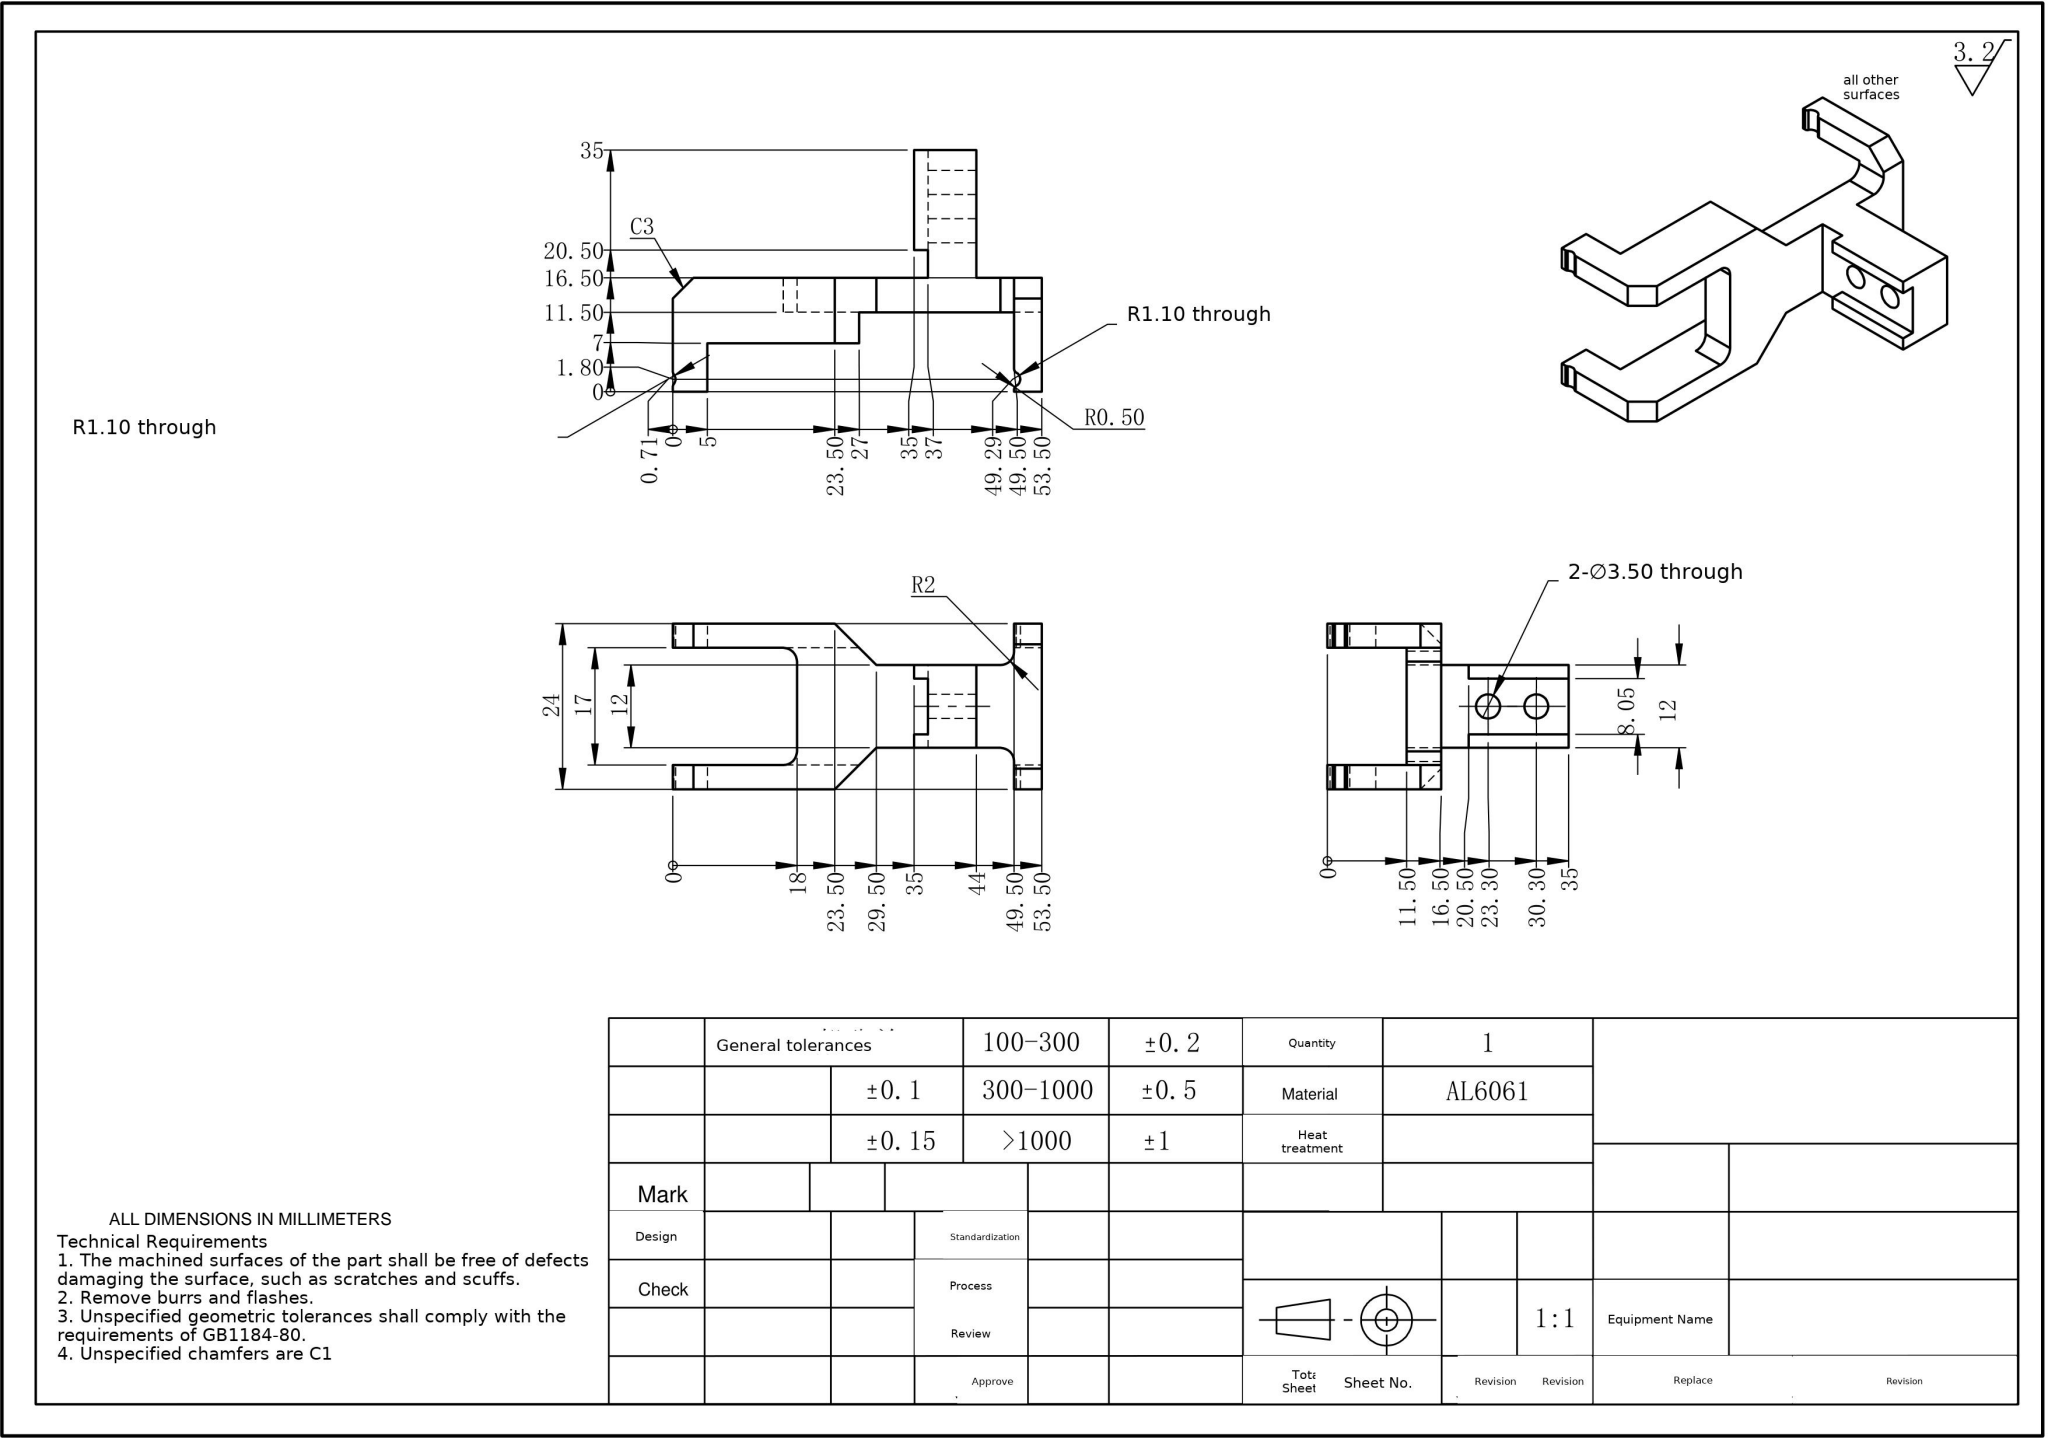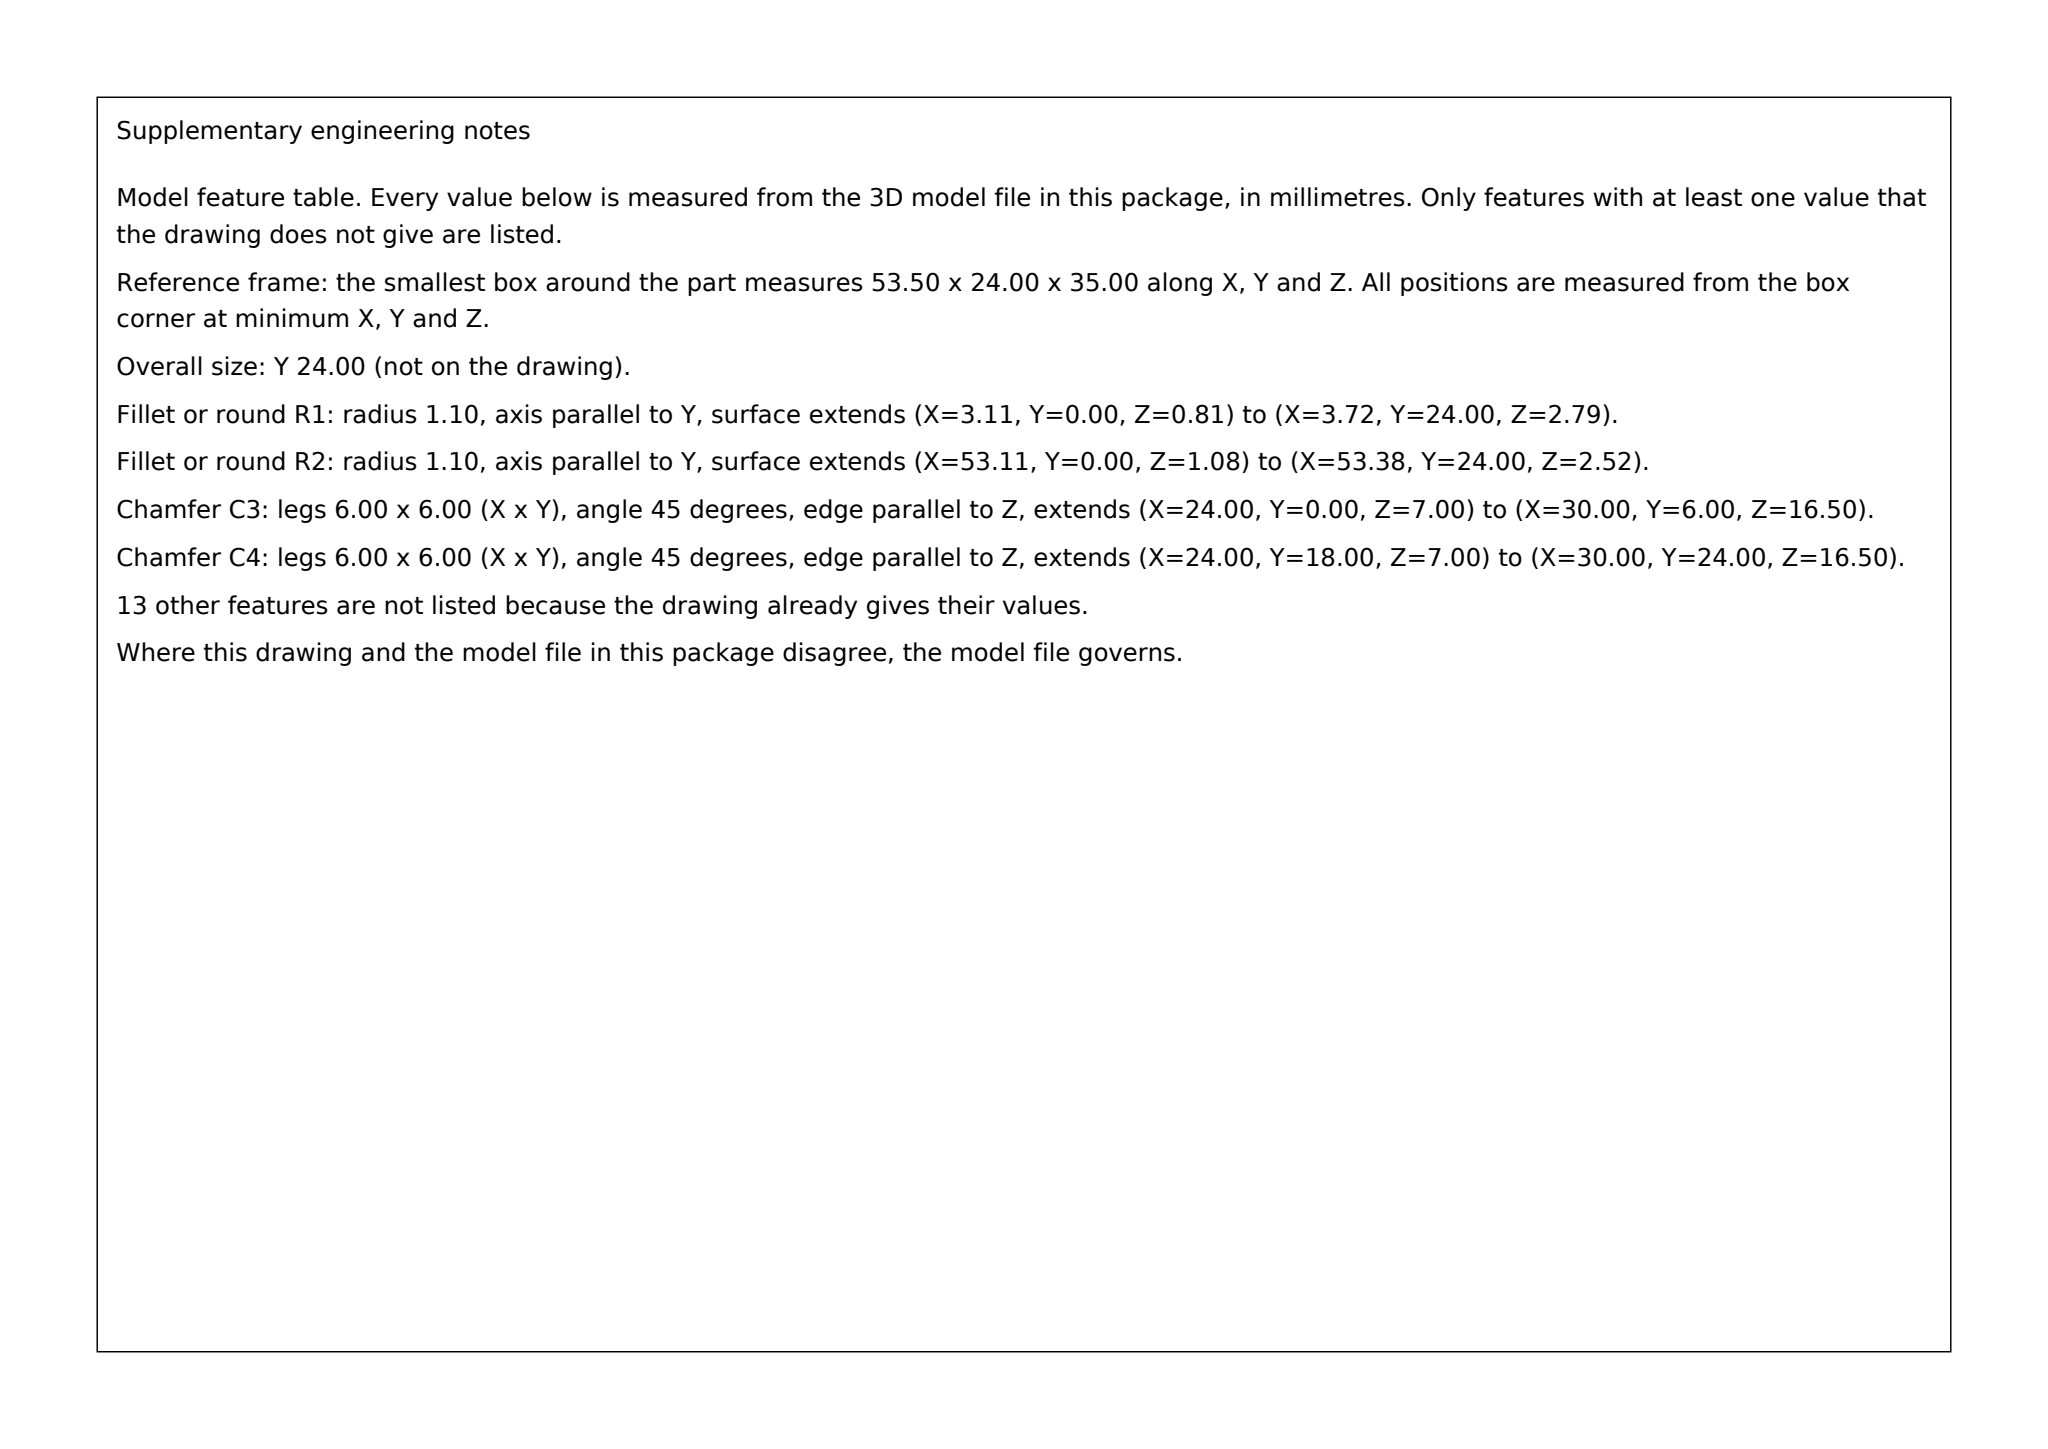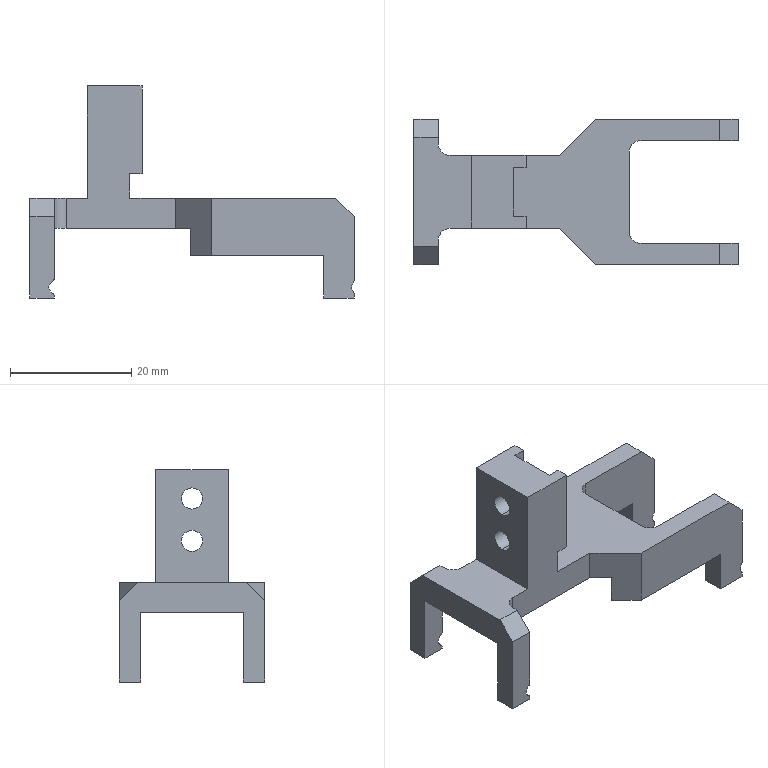Part | SolidWorks | mm | 1 solid | 66 faces | box 53.5 x 24 x 35 mm | volume 6342 mm3 | plane 46 | cylinder 20 | commonest cylinder face diameters 1 x8 3.5 x4 2.2 x4 4 x4